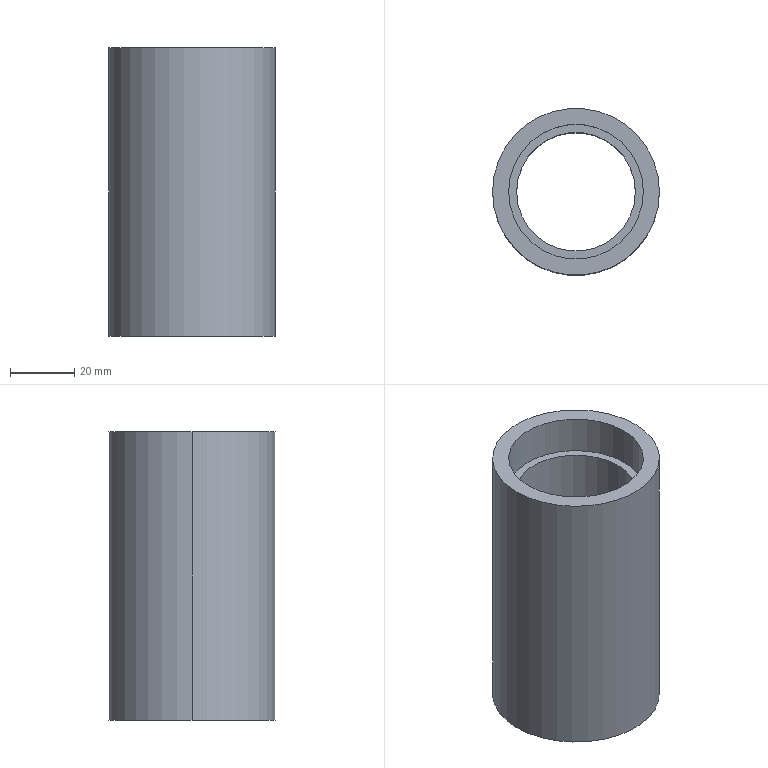Component | SolidWorks | -SmallRollerAssembly-1_-SmallPulley-1 | 1 solid | 12 faces | box 52 x 52 x 90 mm | volume 86920 mm3 | cylinder 8 | plane 4 | commonest cylinder face diameters 42 x4 37 x2 52 x2
build123d program:
from build123d import *


with BuildPart() as part:
    # Sketch1 → Revolve1 (revolve)
    with BuildSketch(Plane.XY, mode=Mode.PRIVATE) as revolve1_sk:
        Polygon((0, 26), (0, 21), (12, 21), (12, 18.5), (78, 18.5), (78, 21), (90, 21), (90, 26), align=None)
    revolve(revolve1_sk.sketch.rotate(Axis((-767.485, 0, 0), (1, 0, 0)), 90), axis=Axis((-767.485, 0, 0), (1, 0, 0)))


solid = part.part

# Placed as in the assembly
solid = solid.moved(Location((-45, 1121, 135), (0, 90, 0)))
STEP:
#1=CARTESIAN_POINT('',(-2.598,44.134,1.772));
#2=VERTEX_POINT('',#1);
#3=CARTESIAN_POINT('',(-0.9449,44.134,1.772));
#4=VERTEX_POINT('',#3);
#5=CARTESIAN_POINT('',(-1.772,44.134,1.772));
#6=DIRECTION('',(-0.,0.,1.));
#7=DIRECTION('',(1.,0.,0.));
#8=AXIS2_PLACEMENT_3D('',#5,#6,#7);
#9=CIRCLE('',#8,0.8268);
#10=EDGE_CURVE('',#2,#4,#9,.T.);
#11=ORIENTED_EDGE('',*,*,#10,.F.);
#12=CARTESIAN_POINT('',(-2.598,44.134,2.244));
#13=VERTEX_POINT('',#12);
#14=CARTESIAN_POINT('',(-2.598,44.134,35.531));
#15=DIRECTION('',(-0.,0.,1.));
#16=VECTOR('',#15,39.37);
#17=LINE('',#14,#16);
#18=EDGE_CURVE('',#2,#13,#17,.T.);
#19=ORIENTED_EDGE('',*,*,#18,.T.);
#20=CARTESIAN_POINT('',(-0.9449,44.134,2.244));
#21=VERTEX_POINT('',#20);
#22=CARTESIAN_POINT('',(-1.772,44.134,2.244));
#23=DIRECTION('',(-0.,0.,1.));
#24=DIRECTION('',(1.,0.,0.));
#25=AXIS2_PLACEMENT_3D('',#22,#23,#24);
#26=CIRCLE('',#25,0.8268);
#27=EDGE_CURVE('',#13,#21,#26,.T.);
#28=ORIENTED_EDGE('',*,*,#27,.T.);
#29=CARTESIAN_POINT('',(-0.9449,44.134,35.531));
#30=DIRECTION('',(-0.,0.,1.));
#31=VECTOR('',#30,39.37);
#32=LINE('',#29,#31);
#33=EDGE_CURVE('',#4,#21,#32,.T.);
#34=ORIENTED_EDGE('',*,*,#33,.F.);
#35=EDGE_LOOP('',(#11,#19,#28,#34));
#36=FACE_OUTER_BOUND('',#35,.T.);
#37=CARTESIAN_POINT('',(-1.772,44.134,35.531));
#38=DIRECTION('',(-0.,0.,1.));
#39=DIRECTION('',(1.,0.,0.));
#40=AXIS2_PLACEMENT_3D('',#37,#38,#39);
#41=CYLINDRICAL_SURFACE('',#40,0.8268);
#42=ADVANCED_FACE('',(#36),#41,.F.);
#43=CARTESIAN_POINT('',(-2.5,44.134,2.244));
#44=VERTEX_POINT('',#43);
#45=CARTESIAN_POINT('',(-1.043,44.134,2.244));
#46=VERTEX_POINT('',#45);
#47=CARTESIAN_POINT('',(-1.772,44.134,2.244));
#48=DIRECTION('',(-0.,0.,1.));
#49=DIRECTION('',(1.,0.,0.));
#50=AXIS2_PLACEMENT_3D('',#47,#48,#49);
#51=CIRCLE('',#50,0.7283);
#52=EDGE_CURVE('',#44,#46,#51,.T.);
#53=ORIENTED_EDGE('',*,*,#52,.F.);
#54=CARTESIAN_POINT('',(-2.5,44.134,4.843));
#55=VERTEX_POINT('',#54);
#56=CARTESIAN_POINT('',(-2.5,44.134,35.531));
#57=DIRECTION('',(-0.,0.,1.));
#58=VECTOR('',#57,39.37);
#59=LINE('',#56,#58);
#60=EDGE_CURVE('',#44,#55,#59,.T.);
#61=ORIENTED_EDGE('',*,*,#60,.T.);
#62=CARTESIAN_POINT('',(-1.043,44.134,4.843));
#63=VERTEX_POINT('',#62);
#64=CARTESIAN_POINT('',(-1.772,44.134,4.843));
#65=DIRECTION('',(-0.,0.,1.));
#66=DIRECTION('',(1.,0.,0.));
#67=AXIS2_PLACEMENT_3D('',#64,#65,#66);
#68=CIRCLE('',#67,0.7283);
#69=EDGE_CURVE('',#55,#63,#68,.T.);
#70=ORIENTED_EDGE('',*,*,#69,.T.);
#71=CARTESIAN_POINT('',(-1.043,44.134,35.531));
#72=DIRECTION('',(-0.,0.,1.));
#73=VECTOR('',#72,39.37);
#74=LINE('',#71,#73);
#75=EDGE_CURVE('',#46,#63,#74,.T.);
#76=ORIENTED_EDGE('',*,*,#75,.F.);
#77=EDGE_LOOP('',(#53,#61,#70,#76));
#78=FACE_OUTER_BOUND('',#77,.T.);
#79=CARTESIAN_POINT('',(-1.772,44.134,35.531));
#80=DIRECTION('',(-0.,0.,1.));
#81=DIRECTION('',(1.,0.,0.));
#82=AXIS2_PLACEMENT_3D('',#79,#80,#81);
#83=CYLINDRICAL_SURFACE('',#82,0.7283);
#84=ADVANCED_FACE('',(#78),#83,.F.);
#85=CARTESIAN_POINT('',(-2.598,44.134,4.843));
#86=VERTEX_POINT('',#85);
#87=CARTESIAN_POINT('',(-0.9449,44.134,4.843));
#88=VERTEX_POINT('',#87);
#89=CARTESIAN_POINT('',(-1.772,44.134,4.843));
#90=DIRECTION('',(-0.,0.,1.));
#91=DIRECTION('',(1.,0.,0.));
#92=AXIS2_PLACEMENT_3D('',#89,#90,#91);
#93=CIRCLE('',#92,0.8268);
#94=EDGE_CURVE('',#86,#88,#93,.T.);
#95=ORIENTED_EDGE('',*,*,#94,.F.);
#96=CARTESIAN_POINT('',(-2.598,44.134,5.315));
#97=VERTEX_POINT('',#96);
#98=CARTESIAN_POINT('',(-2.598,44.134,35.531));
#99=DIRECTION('',(-0.,0.,1.));
#100=VECTOR('',#99,39.37);
#101=LINE('',#98,#100);
#102=EDGE_CURVE('',#86,#97,#101,.T.);
#103=ORIENTED_EDGE('',*,*,#102,.T.);
#104=CARTESIAN_POINT('',(-0.9449,44.134,5.315));
#105=VERTEX_POINT('',#104);
#106=CARTESIAN_POINT('',(-1.772,44.134,5.315));
#107=DIRECTION('',(-0.,0.,1.));
#108=DIRECTION('',(1.,0.,0.));
#109=AXIS2_PLACEMENT_3D('',#106,#107,#108);
#110=CIRCLE('',#109,0.8268);
#111=EDGE_CURVE('',#97,#105,#110,.T.);
#112=ORIENTED_EDGE('',*,*,#111,.T.);
#113=CARTESIAN_POINT('',(-0.9449,44.134,35.531));
#114=DIRECTION('',(-0.,0.,1.));
#115=VECTOR('',#114,39.37);
#116=LINE('',#113,#115);
#117=EDGE_CURVE('',#88,#105,#116,.T.);
#118=ORIENTED_EDGE('',*,*,#117,.F.);
#119=EDGE_LOOP('',(#95,#103,#112,#118));
#120=FACE_OUTER_BOUND('',#119,.T.);
#121=CARTESIAN_POINT('',(-1.772,44.134,35.531));
#122=DIRECTION('',(-0.,0.,1.));
#123=DIRECTION('',(1.,0.,0.));
#124=AXIS2_PLACEMENT_3D('',#121,#122,#123);
#125=CYLINDRICAL_SURFACE('',#124,0.8268);
#126=ADVANCED_FACE('',(#120),#125,.F.);
#127=CARTESIAN_POINT('',(-0.748,44.134,1.772));
#128=VERTEX_POINT('',#127);
#129=CARTESIAN_POINT('',(-2.795,44.134,1.772));
#130=VERTEX_POINT('',#129);
#131=CARTESIAN_POINT('',(-1.772,44.134,1.772));
#132=DIRECTION('',(-0.,0.,1.));
#133=DIRECTION('',(1.,0.,0.));
#134=AXIS2_PLACEMENT_3D('',#131,#132,#133);
#135=CIRCLE('',#134,1.024);
#136=EDGE_CURVE('',#128,#130,#135,.T.);
#137=ORIENTED_EDGE('',*,*,#136,.T.);
#138=CARTESIAN_POINT('',(-2.795,44.134,5.315));
#139=VERTEX_POINT('',#138);
#140=CARTESIAN_POINT('',(-2.795,44.134,35.531));
#141=DIRECTION('',(-0.,0.,1.));
#142=VECTOR('',#141,39.37);
#143=LINE('',#140,#142);
#144=EDGE_CURVE('',#130,#139,#143,.T.);
#145=ORIENTED_EDGE('',*,*,#144,.T.);
#146=CARTESIAN_POINT('',(-0.748,44.134,5.315));
#147=VERTEX_POINT('',#146);
#148=CARTESIAN_POINT('',(-1.772,44.134,5.315));
#149=DIRECTION('',(-0.,0.,1.));
#150=DIRECTION('',(1.,0.,0.));
#151=AXIS2_PLACEMENT_3D('',#148,#149,#150);
#152=CIRCLE('',#151,1.024);
#153=EDGE_CURVE('',#147,#139,#152,.T.);
#154=ORIENTED_EDGE('',*,*,#153,.F.);
#155=CARTESIAN_POINT('',(-0.748,44.134,35.531));
#156=DIRECTION('',(-0.,0.,1.));
#157=VECTOR('',#156,39.37);
#158=LINE('',#155,#157);
#159=EDGE_CURVE('',#128,#147,#158,.T.);
#160=ORIENTED_EDGE('',*,*,#159,.F.);
#161=EDGE_LOOP('',(#137,#145,#154,#160));
#162=FACE_OUTER_BOUND('',#161,.T.);
#163=CARTESIAN_POINT('',(-1.772,44.134,35.531));
#164=DIRECTION('',(-0.,0.,1.));
#165=DIRECTION('',(1.,0.,0.));
#166=AXIS2_PLACEMENT_3D('',#163,#164,#165);
#167=CYLINDRICAL_SURFACE('',#166,1.024);
#168=ADVANCED_FACE('',(#162),#167,.T.);
#169=ORIENTED_EDGE('',*,*,#144,.F.);
#170=CARTESIAN_POINT('',(-1.772,44.134,1.772));
#171=DIRECTION('',(-0.,0.,1.));
#172=DIRECTION('',(1.,0.,0.));
#173=AXIS2_PLACEMENT_3D('',#170,#171,#172);
#174=CIRCLE('',#173,1.024);
#175=EDGE_CURVE('',#130,#128,#174,.T.);
#176=ORIENTED_EDGE('',*,*,#175,.T.);
#177=ORIENTED_EDGE('',*,*,#159,.T.);
#178=CARTESIAN_POINT('',(-1.772,44.134,5.315));
#179=DIRECTION('',(-0.,0.,1.));
#180=DIRECTION('',(1.,0.,0.));
#181=AXIS2_PLACEMENT_3D('',#178,#179,#180);
#182=CIRCLE('',#181,1.024);
#183=EDGE_CURVE('',#139,#147,#182,.T.);
#184=ORIENTED_EDGE('',*,*,#183,.F.);
#185=EDGE_LOOP('',(#169,#176,#177,#184));
#186=FACE_OUTER_BOUND('',#185,.T.);
#187=CARTESIAN_POINT('',(-1.772,44.134,35.531));
#188=DIRECTION('',(-0.,0.,1.));
#189=DIRECTION('',(1.,0.,0.));
#190=AXIS2_PLACEMENT_3D('',#187,#188,#189);
#191=CYLINDRICAL_SURFACE('',#190,1.024);
#192=ADVANCED_FACE('',(#186),#191,.T.);
#193=CARTESIAN_POINT('',(-1.772,44.134,5.315));
#194=DIRECTION('',(-0.,0.,1.));
#195=DIRECTION('',(1.,0.,0.));
#196=AXIS2_PLACEMENT_3D('',#193,#194,#195);
#197=CIRCLE('',#196,0.8268);
#198=EDGE_CURVE('',#105,#97,#197,.T.);
#199=ORIENTED_EDGE('',*,*,#198,.F.);
#200=ORIENTED_EDGE('',*,*,#111,.F.);
#201=EDGE_LOOP('',(#199,#200));
#202=FACE_BOUND('',#201,.T.);
#203=ORIENTED_EDGE('',*,*,#153,.T.);
#204=ORIENTED_EDGE('',*,*,#183,.T.);
#205=EDGE_LOOP('',(#203,#204));
#206=FACE_OUTER_BOUND('',#205,.T.);
#207=CARTESIAN_POINT('',(-1.772,45.157,5.315));
#208=DIRECTION('',(0.,0.,-1.));
#209=DIRECTION('',(-1.,0.,-0.));
#210=AXIS2_PLACEMENT_3D('',#207,#208,#209);
#211=PLANE('',#210);
#212=ADVANCED_FACE('',(#202,#206),#211,.F.);
#213=ORIENTED_EDGE('',*,*,#102,.F.);
#214=CARTESIAN_POINT('',(-1.772,44.134,4.843));
#215=DIRECTION('',(-0.,0.,1.));
#216=DIRECTION('',(1.,0.,0.));
#217=AXIS2_PLACEMENT_3D('',#214,#215,#216);
#218=CIRCLE('',#217,0.8268);
#219=EDGE_CURVE('',#88,#86,#218,.T.);
#220=ORIENTED_EDGE('',*,*,#219,.F.);
#221=ORIENTED_EDGE('',*,*,#117,.T.);
#222=ORIENTED_EDGE('',*,*,#198,.T.);
#223=EDGE_LOOP('',(#213,#220,#221,#222));
#224=FACE_OUTER_BOUND('',#223,.T.);
#225=CARTESIAN_POINT('',(-1.772,44.134,35.531));
#226=DIRECTION('',(-0.,0.,1.));
#227=DIRECTION('',(1.,0.,0.));
#228=AXIS2_PLACEMENT_3D('',#225,#226,#227);
#229=CYLINDRICAL_SURFACE('',#228,0.8268);
#230=ADVANCED_FACE('',(#224),#229,.F.);
#231=CARTESIAN_POINT('',(-1.772,44.134,4.843));
#232=DIRECTION('',(-0.,0.,1.));
#233=DIRECTION('',(1.,0.,0.));
#234=AXIS2_PLACEMENT_3D('',#231,#232,#233);
#235=CIRCLE('',#234,0.7283);
#236=EDGE_CURVE('',#63,#55,#235,.T.);
#237=ORIENTED_EDGE('',*,*,#236,.F.);
#238=ORIENTED_EDGE('',*,*,#69,.F.);
#239=EDGE_LOOP('',(#237,#238));
#240=FACE_BOUND('',#239,.T.);
#241=ORIENTED_EDGE('',*,*,#219,.T.);
#242=ORIENTED_EDGE('',*,*,#94,.T.);
#243=EDGE_LOOP('',(#241,#242));
#244=FACE_OUTER_BOUND('',#243,.T.);
#245=CARTESIAN_POINT('',(-1.772,44.961,4.843));
#246=DIRECTION('',(0.,0.,-1.));
#247=DIRECTION('',(-1.,0.,-0.));
#248=AXIS2_PLACEMENT_3D('',#245,#246,#247);
#249=PLANE('',#248);
#250=ADVANCED_FACE('',(#240,#244),#249,.F.);
#251=ORIENTED_EDGE('',*,*,#60,.F.);
#252=CARTESIAN_POINT('',(-1.772,44.134,2.244));
#253=DIRECTION('',(-0.,0.,1.));
#254=DIRECTION('',(1.,0.,0.));
#255=AXIS2_PLACEMENT_3D('',#252,#253,#254);
#256=CIRCLE('',#255,0.7283);
#257=EDGE_CURVE('',#46,#44,#256,.T.);
#258=ORIENTED_EDGE('',*,*,#257,.F.);
#259=ORIENTED_EDGE('',*,*,#75,.T.);
#260=ORIENTED_EDGE('',*,*,#236,.T.);
#261=EDGE_LOOP('',(#251,#258,#259,#260));
#262=FACE_OUTER_BOUND('',#261,.T.);
#263=CARTESIAN_POINT('',(-1.772,44.134,35.531));
#264=DIRECTION('',(-0.,0.,1.));
#265=DIRECTION('',(1.,0.,0.));
#266=AXIS2_PLACEMENT_3D('',#263,#264,#265);
#267=CYLINDRICAL_SURFACE('',#266,0.7283);
#268=ADVANCED_FACE('',(#262),#267,.F.);
#269=CARTESIAN_POINT('',(-1.772,44.134,2.244));
#270=DIRECTION('',(-0.,0.,1.));
#271=DIRECTION('',(1.,0.,0.));
#272=AXIS2_PLACEMENT_3D('',#269,#270,#271);
#273=CIRCLE('',#272,0.8268);
#274=EDGE_CURVE('',#21,#13,#273,.T.);
#275=ORIENTED_EDGE('',*,*,#274,.F.);
#276=ORIENTED_EDGE('',*,*,#27,.F.);
#277=EDGE_LOOP('',(#275,#276));
#278=FACE_OUTER_BOUND('',#277,.T.);
#279=ORIENTED_EDGE('',*,*,#257,.T.);
#280=ORIENTED_EDGE('',*,*,#52,.T.);
#281=EDGE_LOOP('',(#279,#280));
#282=FACE_BOUND('',#281,.T.);
#283=CARTESIAN_POINT('',(-1.772,44.862,2.244));
#284=DIRECTION('',(-0.,0.,1.));
#285=DIRECTION('',(1.,0.,0.));
#286=AXIS2_PLACEMENT_3D('',#283,#284,#285);
#287=PLANE('',#286);
#288=ADVANCED_FACE('',(#278,#282),#287,.F.);
#289=ORIENTED_EDGE('',*,*,#18,.F.);
#290=CARTESIAN_POINT('',(-1.772,44.134,1.772));
#291=DIRECTION('',(-0.,0.,1.));
#292=DIRECTION('',(1.,0.,0.));
#293=AXIS2_PLACEMENT_3D('',#290,#291,#292);
#294=CIRCLE('',#293,0.8268);
#295=EDGE_CURVE('',#4,#2,#294,.T.);
#296=ORIENTED_EDGE('',*,*,#295,.F.);
#297=ORIENTED_EDGE('',*,*,#33,.T.);
#298=ORIENTED_EDGE('',*,*,#274,.T.);
#299=EDGE_LOOP('',(#289,#296,#297,#298));
#300=FACE_OUTER_BOUND('',#299,.T.);
#301=CARTESIAN_POINT('',(-1.772,44.134,35.531));
#302=DIRECTION('',(-0.,0.,1.));
#303=DIRECTION('',(1.,0.,0.));
#304=AXIS2_PLACEMENT_3D('',#301,#302,#303);
#305=CYLINDRICAL_SURFACE('',#304,0.8268);
#306=ADVANCED_FACE('',(#300),#305,.F.);
#307=ORIENTED_EDGE('',*,*,#136,.F.);
#308=ORIENTED_EDGE('',*,*,#175,.F.);
#309=EDGE_LOOP('',(#307,#308));
#310=FACE_OUTER_BOUND('',#309,.T.);
#311=ORIENTED_EDGE('',*,*,#295,.T.);
#312=ORIENTED_EDGE('',*,*,#10,.T.);
#313=EDGE_LOOP('',(#311,#312));
#314=FACE_BOUND('',#313,.T.);
#315=CARTESIAN_POINT('',(-1.772,44.961,1.772));
#316=DIRECTION('',(-0.,0.,1.));
#317=DIRECTION('',(1.,0.,0.));
#318=AXIS2_PLACEMENT_3D('',#315,#316,#317);
#319=PLANE('',#318);
#320=ADVANCED_FACE('',(#310,#314),#319,.F.);
#321=CLOSED_SHELL('',(#42,#84,#126,#168,#192,#212,#230,#250,#268,#288,#306,#320));
#322=MANIFOLD_SOLID_BREP('',#321);
#323=CARTESIAN_POINT('',(0.,0.,0.));
#324=DIRECTION('',(0.,0.,1.));
#325=DIRECTION('',(1.,0.,0.));
#326=AXIS2_PLACEMENT_3D('',#323,#324,#325);
#327=(LENGTH_UNIT()NAMED_UNIT(*)SI_UNIT($,.METRE.));
#328=LENGTH_MEASURE_WITH_UNIT(LENGTH_MEASURE(0.0254),#327);
#329=DIMENSIONAL_EXPONENTS(1.,0.,0.,0.,0.,0.,0.);
#330=(CONVERSION_BASED_UNIT('',#328)LENGTH_UNIT()NAMED_UNIT(#329));
#331=UNCERTAINTY_MEASURE_WITH_UNIT(LENGTH_MEASURE(0.00001),#330,'','');
#332=(NAMED_UNIT(*)PLANE_ANGLE_UNIT()SI_UNIT($,.RADIAN.));
#333=(NAMED_UNIT(*)SI_UNIT($,.STERADIAN.)SOLID_ANGLE_UNIT());
#334=(GEOMETRIC_REPRESENTATION_CONTEXT(3)GLOBAL_UNCERTAINTY_ASSIGNED_CONTEXT((#331))GLOBAL_UNIT_ASSIGNED_CONTEXT((#330,#332,#333))REPRESENTATION_CONTEXT('',''));
#335=ADVANCED_BREP_SHAPE_REPRESENTATION('',(#322,#326),#334);
#336=COLOUR_RGB('',0.7922,0.8196,0.9333);
#337=FILL_AREA_STYLE_COLOUR('',#336);
#338=FILL_AREA_STYLE('',(#337));
#339=SURFACE_STYLE_FILL_AREA(#338);
#340=SURFACE_SIDE_STYLE('',(#339));
#341=SURFACE_STYLE_USAGE(.BOTH.,#340);
#342=PRESENTATION_STYLE_ASSIGNMENT((#341));
#343=STYLED_ITEM('',(#342),#322);
#344=PRESENTATION_LAYER_ASSIGNMENT('','',(#343));
#345=(LENGTH_UNIT()NAMED_UNIT(*)SI_UNIT($,.METRE.));
#346=LENGTH_MEASURE_WITH_UNIT(LENGTH_MEASURE(0.0254),#345);
#347=DIMENSIONAL_EXPONENTS(1.,0.,0.,0.,0.,0.,0.);
#348=(CONVERSION_BASED_UNIT('',#346)LENGTH_UNIT()NAMED_UNIT(#347));
#349=UNCERTAINTY_MEASURE_WITH_UNIT(LENGTH_MEASURE(0.00001),#348,'','');
#350=(NAMED_UNIT(*)PLANE_ANGLE_UNIT()SI_UNIT($,.RADIAN.));
#351=(NAMED_UNIT(*)SI_UNIT($,.STERADIAN.)SOLID_ANGLE_UNIT());
#352=(GEOMETRIC_REPRESENTATION_CONTEXT(3)GLOBAL_UNCERTAINTY_ASSIGNED_CONTEXT((#349))GLOBAL_UNIT_ASSIGNED_CONTEXT((#348,#350,#351))REPRESENTATION_CONTEXT('',''));
#353=MECHANICAL_DESIGN_GEOMETRIC_PRESENTATION_REPRESENTATION('',(#343),#352);